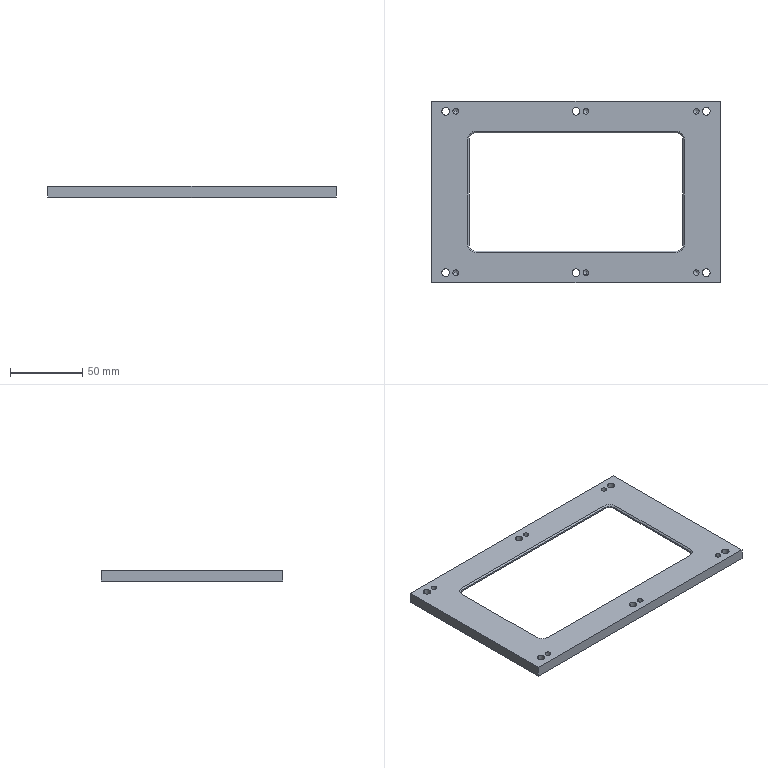CAM job | Mastercam | mm | 14 operations | part box 200 x 126 x 8
1. Facing | 24 - 100 平铣刀
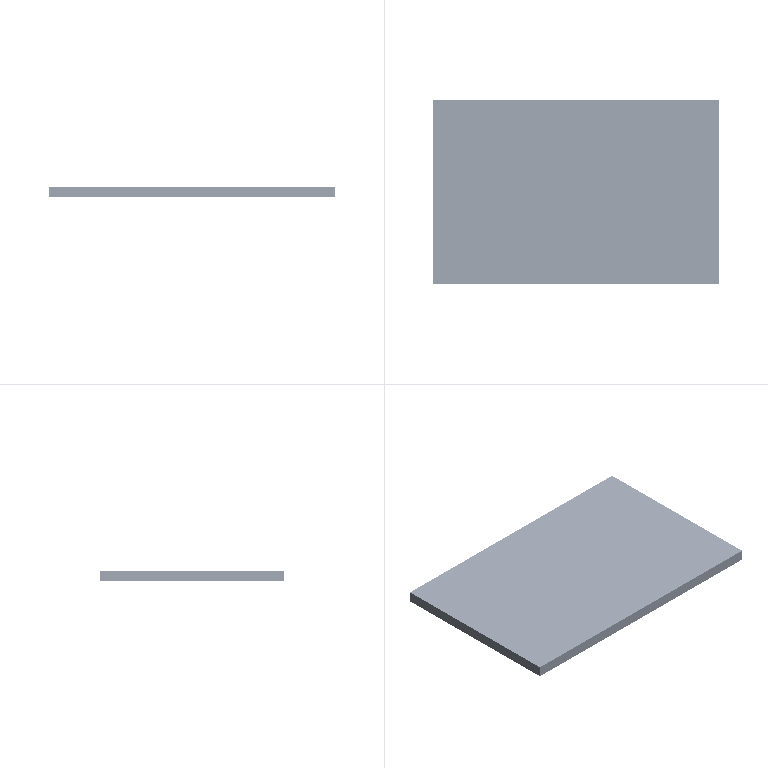2. Contour (Ramp) | 10 - 10 平铣刀
3. Contour (2D) | 10 - 10 平铣刀
4. 2D High Speed (2D Area Mill) | 10 - 10 平铣刀
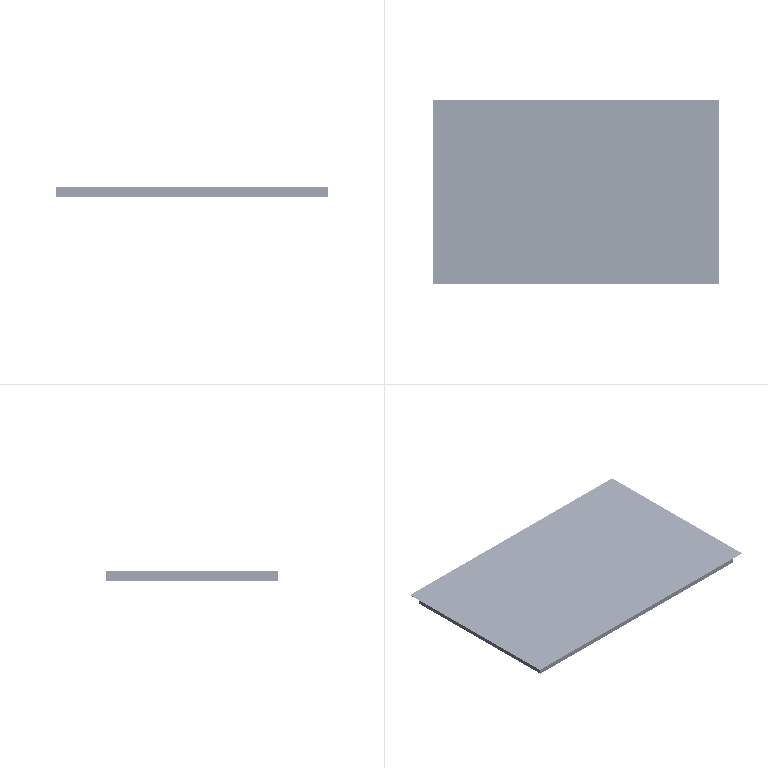5. Contour (2D) | 10 - 10 平铣刀
6. Contour (Ramp) | 4 - 4 平铣刀
7. Contour (2D) | 3 - 3 平铣刀
8. Contour (2D chamfer) | 7 - 4 倒角刀
9. Contour (2D chamfer) | 7 - 4 倒角刀
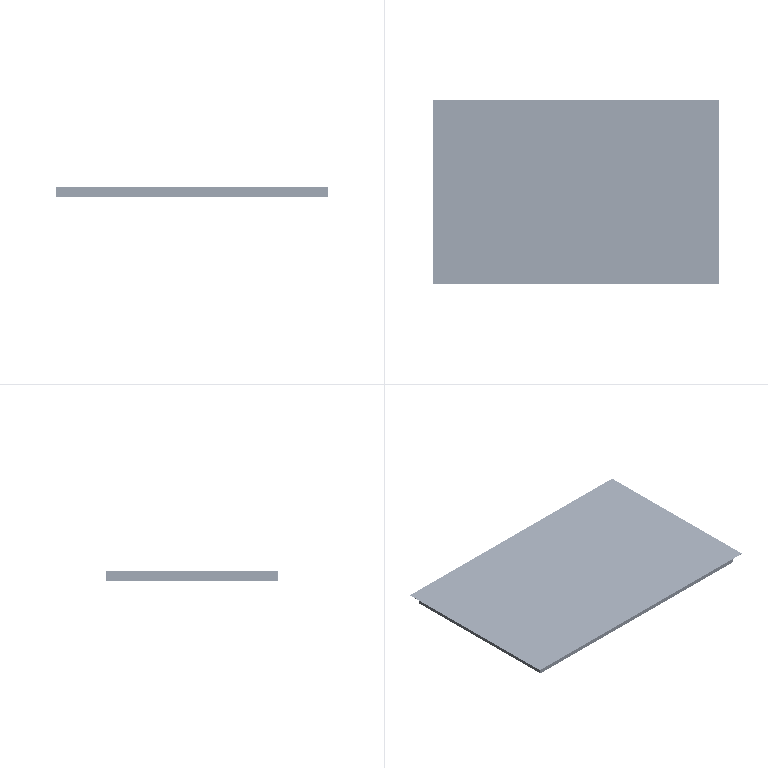10. Contour (2D chamfer) | 7 - 4 倒角刀
11. Drill/Counterbore | 7 - 4 倒角刀
12. Contour (2D chamfer) | 7 - 4 倒角刀
13. Contour (2D chamfer) | 7 - 4 倒角刀
14. Drill/Counterbore | 7 - 4 倒角刀